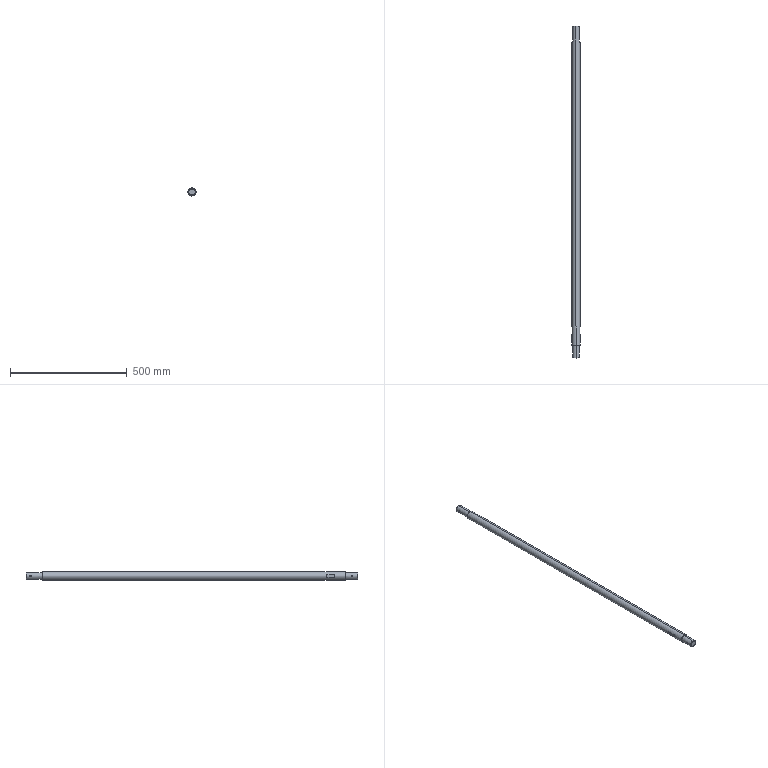Component | SolidWorks | YC1-250-04BalancerAssembly#16673-1_YC1-250-04-06TieRodAxis#16673-1 | 1 solid | 28 faces | box 35 x 1424 x 35 mm | volume 1335790 mm3 | cylinder 10 | plane 10 | cone 8 | commonest cylinder face diameters 30 x4 6 x4 35 x2 | material Plain Carbon Steel
STEP:
#1=COLOUR_RGB('',0.7922,0.8196,0.9333);
#2=FILL_AREA_STYLE_COLOUR('',#1);
#3=FILL_AREA_STYLE('',(#2));
#4=SURFACE_STYLE_FILL_AREA(#3);
#5=SURFACE_SIDE_STYLE('',(#4));
#6=SURFACE_STYLE_USAGE(.BOTH.,#5);
#7=PRESENTATION_STYLE_ASSIGNMENT((#6));
#8=CARTESIAN_POINT('',(-18.689,112.992,-0.1181));
#9=VERTEX_POINT('',#8);
#10=CARTESIAN_POINT('',(-18.689,112.992,0.1181));
#11=VERTEX_POINT('',#10);
#12=CARTESIAN_POINT('',(-18.689,112.992,-0.1181));
#13=CARTESIAN_POINT('',(-18.689,113.,-0.1181));
#14=CARTESIAN_POINT('',(-18.689,113.008,-0.1173));
#15=CARTESIAN_POINT('',(-18.69,113.023,-0.1143));
#16=CARTESIAN_POINT('',(-18.69,113.03,-0.112));
#17=CARTESIAN_POINT('',(-18.691,113.045,-0.1061));
#18=CARTESIAN_POINT('',(-18.692,113.051,-0.1025));
#19=CARTESIAN_POINT('',(-18.693,113.064,-0.09392));
#20=CARTESIAN_POINT('',(-18.694,113.07,-0.08895));
#21=CARTESIAN_POINT('',(-18.696,113.081,-0.07808));
#22=CARTESIAN_POINT('',(-18.696,113.086,-0.07215));
#23=CARTESIAN_POINT('',(-18.698,113.095,-0.05925));
#24=CARTESIAN_POINT('',(-18.699,113.098,-0.05241));
#25=CARTESIAN_POINT('',(-18.7,113.104,-0.03821));
#26=CARTESIAN_POINT('',(-18.7,113.106,-0.03075));
#27=CARTESIAN_POINT('',(-18.701,113.109,-0.01549));
#28=CARTESIAN_POINT('',(-18.701,113.11,-0.007819));
#29=CARTESIAN_POINT('',(-18.701,113.11,0.007627));
#30=CARTESIAN_POINT('',(-18.701,113.109,0.01548));
#31=CARTESIAN_POINT('',(-18.7,113.106,0.03064));
#32=CARTESIAN_POINT('',(-18.7,113.104,0.03801));
#33=CARTESIAN_POINT('',(-18.699,113.098,0.05233));
#34=CARTESIAN_POINT('',(-18.698,113.095,0.05922));
#35=CARTESIAN_POINT('',(-18.696,113.086,0.07199));
#36=CARTESIAN_POINT('',(-18.696,113.081,0.07798));
#37=CARTESIAN_POINT('',(-18.694,113.07,0.08896));
#38=CARTESIAN_POINT('',(-18.693,113.064,0.09384));
#39=CARTESIAN_POINT('',(-18.692,113.051,0.1024));
#40=CARTESIAN_POINT('',(-18.691,113.045,0.1061));
#41=CARTESIAN_POINT('',(-18.69,113.03,0.112));
#42=CARTESIAN_POINT('',(-18.69,113.023,0.1143));
#43=CARTESIAN_POINT('',(-18.689,113.008,0.1173));
#44=CARTESIAN_POINT('',(-18.689,113.,0.1181));
#45=CARTESIAN_POINT('',(-18.689,112.992,0.1181));
#46=B_SPLINE_CURVE_WITH_KNOTS('',3,(#12,#13,#14,#15,#16,#17,#18,#19,#20,#21,#22,#23,#24,#25,#26,#27,#28,#29,#30,#31,#32,#33,#34,#35,#36,#37,#38,#39,#40,#41,#42,#43,#44,#45),.UNSPECIFIED.,.F.,.F.,(4,2,2,2,2,2,2,2,2,2,2,2,2,2,2,2,4),(0.,0.0005875,0.001175,0.001763,0.00235,0.002938,0.003525,0.004113,0.0047,0.005288,0.005875,0.006463,0.00705,0.007638,0.008225,0.008813,0.009401),.UNSPECIFIED.);
#47=EDGE_CURVE('',#9,#11,#46,.T.);
#48=ORIENTED_EDGE('',*,*,#47,.T.);
#49=CARTESIAN_POINT('',(-18.689,112.992,0.1181));
#50=CARTESIAN_POINT('',(-18.689,112.984,0.1181));
#51=CARTESIAN_POINT('',(-18.689,112.977,0.1173));
#52=CARTESIAN_POINT('',(-18.69,112.961,0.1143));
#53=CARTESIAN_POINT('',(-18.69,112.954,0.112));
#54=CARTESIAN_POINT('',(-18.691,112.94,0.1061));
#55=CARTESIAN_POINT('',(-18.692,112.933,0.1025));
#56=CARTESIAN_POINT('',(-18.693,112.92,0.09392));
#57=CARTESIAN_POINT('',(-18.694,112.914,0.08895));
#58=CARTESIAN_POINT('',(-18.696,112.903,0.07808));
#59=CARTESIAN_POINT('',(-18.696,112.898,0.07215));
#60=CARTESIAN_POINT('',(-18.698,112.89,0.05925));
#61=CARTESIAN_POINT('',(-18.699,112.886,0.05241));
#62=CARTESIAN_POINT('',(-18.7,112.88,0.03821));
#63=CARTESIAN_POINT('',(-18.7,112.878,0.03075));
#64=CARTESIAN_POINT('',(-18.701,112.875,0.01549));
#65=CARTESIAN_POINT('',(-18.701,112.874,0.007819));
#66=CARTESIAN_POINT('',(-18.701,112.874,-0.007627));
#67=CARTESIAN_POINT('',(-18.701,112.875,-0.01548));
#68=CARTESIAN_POINT('',(-18.7,112.878,-0.03064));
#69=CARTESIAN_POINT('',(-18.7,112.88,-0.03801));
#70=CARTESIAN_POINT('',(-18.699,112.886,-0.05233));
#71=CARTESIAN_POINT('',(-18.698,112.89,-0.05922));
#72=CARTESIAN_POINT('',(-18.696,112.898,-0.07199));
#73=CARTESIAN_POINT('',(-18.696,112.903,-0.07798));
#74=CARTESIAN_POINT('',(-18.694,112.914,-0.08896));
#75=CARTESIAN_POINT('',(-18.693,112.92,-0.09384));
#76=CARTESIAN_POINT('',(-18.692,112.933,-0.1024));
#77=CARTESIAN_POINT('',(-18.691,112.94,-0.1061));
#78=CARTESIAN_POINT('',(-18.69,112.954,-0.112));
#79=CARTESIAN_POINT('',(-18.69,112.961,-0.1143));
#80=CARTESIAN_POINT('',(-18.689,112.976,-0.1173));
#81=CARTESIAN_POINT('',(-18.689,112.984,-0.1181));
#82=CARTESIAN_POINT('',(-18.689,112.992,-0.1181));
#83=B_SPLINE_CURVE_WITH_KNOTS('',3,(#49,#50,#51,#52,#53,#54,#55,#56,#57,#58,#59,#60,#61,#62,#63,#64,#65,#66,#67,#68,#69,#70,#71,#72,#73,#74,#75,#76,#77,#78,#79,#80,#81,#82),.UNSPECIFIED.,.F.,.F.,(4,2,2,2,2,2,2,2,2,2,2,2,2,2,2,2,4),(0.009401,0.009988,0.01058,0.01116,0.01175,0.01234,0.01293,0.01351,0.0141,0.01469,0.01528,0.01586,0.01645,0.01704,0.01763,0.01821,0.0188),.UNSPECIFIED.);
#84=EDGE_CURVE('',#11,#9,#83,.T.);
#85=ORIENTED_EDGE('',*,*,#84,.T.);
#86=EDGE_LOOP('',(#48,#85));
#87=FACE_BOUND('',#86,.T.);
#88=CARTESIAN_POINT('',(-18.11,114.173,0.5906));
#89=VERTEX_POINT('',#88);
#90=CARTESIAN_POINT('',(-18.11,114.173,-0.5906));
#91=VERTEX_POINT('',#90);
#92=CARTESIAN_POINT('',(-18.11,114.173,0.));
#93=DIRECTION('',(0.,-1.,-0.));
#94=DIRECTION('',(0.,0.,1.));
#95=AXIS2_PLACEMENT_3D('',#92,#93,#94);
#96=CIRCLE('',#95,0.5906);
#97=EDGE_CURVE('',#89,#91,#96,.T.);
#98=ORIENTED_EDGE('',*,*,#97,.T.);
#99=CARTESIAN_POINT('',(-18.11,112.087,-0.5906));
#100=VERTEX_POINT('',#99);
#101=CARTESIAN_POINT('',(-18.11,112.008,-0.5906));
#102=DIRECTION('',(0.,-1.,-0.));
#103=VECTOR('',#102,39.37);
#104=LINE('',#101,#103);
#105=EDGE_CURVE('',#91,#100,#104,.T.);
#106=ORIENTED_EDGE('',*,*,#105,.T.);
#107=CARTESIAN_POINT('',(-18.11,112.087,0.5906));
#108=VERTEX_POINT('',#107);
#109=CARTESIAN_POINT('',(-18.11,112.087,0.));
#110=DIRECTION('',(-0.,1.,0.));
#111=DIRECTION('',(0.,0.,1.));
#112=AXIS2_PLACEMENT_3D('',#109,#110,#111);
#113=CIRCLE('',#112,0.5906);
#114=EDGE_CURVE('',#100,#108,#113,.T.);
#115=ORIENTED_EDGE('',*,*,#114,.T.);
#116=CARTESIAN_POINT('',(-18.11,112.008,0.5906));
#117=DIRECTION('',(0.,-1.,-0.));
#118=VECTOR('',#117,39.37);
#119=LINE('',#116,#118);
#120=EDGE_CURVE('',#89,#108,#119,.T.);
#121=ORIENTED_EDGE('',*,*,#120,.F.);
#122=EDGE_LOOP('',(#98,#106,#115,#121));
#123=FACE_OUTER_BOUND('',#122,.T.);
#124=CARTESIAN_POINT('',(-18.11,112.008,0.));
#125=DIRECTION('',(0.,-1.,-0.));
#126=DIRECTION('',(0.,0.,1.));
#127=AXIS2_PLACEMENT_3D('',#124,#125,#126);
#128=CYLINDRICAL_SURFACE('',#127,0.5906);
#129=ADVANCED_FACE('',(#87,#123),#128,.T.);
#130=ORIENTED_EDGE('',*,*,#84,.F.);
#131=CARTESIAN_POINT('',(-17.532,112.992,0.1181));
#132=VERTEX_POINT('',#131);
#133=CARTESIAN_POINT('',(-17.52,112.992,0.1181));
#134=DIRECTION('',(1.,0.,-0.));
#135=VECTOR('',#134,39.37);
#136=LINE('',#133,#135);
#137=EDGE_CURVE('',#11,#132,#136,.T.);
#138=ORIENTED_EDGE('',*,*,#137,.T.);
#139=CARTESIAN_POINT('',(-17.532,112.992,-0.1181));
#140=VERTEX_POINT('',#139);
#141=CARTESIAN_POINT('',(-17.532,112.992,-0.1181));
#142=CARTESIAN_POINT('',(-17.532,112.984,-0.1181));
#143=CARTESIAN_POINT('',(-17.531,112.977,-0.1173));
#144=CARTESIAN_POINT('',(-17.531,112.961,-0.1143));
#145=CARTESIAN_POINT('',(-17.53,112.954,-0.112));
#146=CARTESIAN_POINT('',(-17.529,112.94,-0.1061));
#147=CARTESIAN_POINT('',(-17.529,112.933,-0.1025));
#148=CARTESIAN_POINT('',(-17.527,112.92,-0.09392));
#149=CARTESIAN_POINT('',(-17.526,112.914,-0.08895));
#150=CARTESIAN_POINT('',(-17.525,112.903,-0.07808));
#151=CARTESIAN_POINT('',(-17.524,112.898,-0.07215));
#152=CARTESIAN_POINT('',(-17.523,112.89,-0.05925));
#153=CARTESIAN_POINT('',(-17.522,112.886,-0.05241));
#154=CARTESIAN_POINT('',(-17.521,112.88,-0.03821));
#155=CARTESIAN_POINT('',(-17.52,112.878,-0.03075));
#156=CARTESIAN_POINT('',(-17.52,112.875,-0.01549));
#157=CARTESIAN_POINT('',(-17.52,112.874,-0.007819));
#158=CARTESIAN_POINT('',(-17.52,112.874,0.007627));
#159=CARTESIAN_POINT('',(-17.52,112.875,0.01548));
#160=CARTESIAN_POINT('',(-17.52,112.878,0.03064));
#161=CARTESIAN_POINT('',(-17.521,112.88,0.03801));
#162=CARTESIAN_POINT('',(-17.522,112.886,0.05233));
#163=CARTESIAN_POINT('',(-17.523,112.89,0.05922));
#164=CARTESIAN_POINT('',(-17.524,112.898,0.07199));
#165=CARTESIAN_POINT('',(-17.525,112.903,0.07798));
#166=CARTESIAN_POINT('',(-17.526,112.914,0.08896));
#167=CARTESIAN_POINT('',(-17.527,112.92,0.09384));
#168=CARTESIAN_POINT('',(-17.529,112.933,0.1024));
#169=CARTESIAN_POINT('',(-17.529,112.94,0.1061));
#170=CARTESIAN_POINT('',(-17.53,112.954,0.112));
#171=CARTESIAN_POINT('',(-17.531,112.961,0.1143));
#172=CARTESIAN_POINT('',(-17.531,112.976,0.1173));
#173=CARTESIAN_POINT('',(-17.532,112.984,0.1181));
#174=CARTESIAN_POINT('',(-17.532,112.992,0.1181));
#175=B_SPLINE_CURVE_WITH_KNOTS('',3,(#141,#142,#143,#144,#145,#146,#147,#148,#149,#150,#151,#152,#153,#154,#155,#156,#157,#158,#159,#160,#161,#162,#163,#164,#165,#166,#167,#168,#169,#170,#171,#172,#173,#174),.UNSPECIFIED.,.F.,.F.,(4,2,2,2,2,2,2,2,2,2,2,2,2,2,2,2,4),(0.,0.0005875,0.001175,0.001763,0.00235,0.002938,0.003525,0.004113,0.0047,0.005288,0.005875,0.006463,0.00705,0.007638,0.008225,0.008813,0.009401),.UNSPECIFIED.);
#176=EDGE_CURVE('',#140,#132,#175,.T.);
#177=ORIENTED_EDGE('',*,*,#176,.F.);
#178=CARTESIAN_POINT('',(-17.52,112.992,-0.1181));
#179=DIRECTION('',(1.,0.,-0.));
#180=VECTOR('',#179,39.37);
#181=LINE('',#178,#180);
#182=EDGE_CURVE('',#9,#140,#181,.T.);
#183=ORIENTED_EDGE('',*,*,#182,.F.);
#184=EDGE_LOOP('',(#130,#138,#177,#183));
#185=FACE_OUTER_BOUND('',#184,.T.);
#186=CARTESIAN_POINT('',(-17.52,112.992,0.));
#187=DIRECTION('',(1.,0.,-0.));
#188=DIRECTION('',(0.,0.,-1.));
#189=AXIS2_PLACEMENT_3D('',#186,#187,#188);
#190=CYLINDRICAL_SURFACE('',#189,0.1181);
#191=ADVANCED_FACE('',(#185),#190,.F.);
#192=CARTESIAN_POINT('',(-18.11,112.008,-0.5118));
#193=VERTEX_POINT('',#192);
#194=CARTESIAN_POINT('',(-18.11,112.008,0.5118));
#195=VERTEX_POINT('',#194);
#196=CARTESIAN_POINT('',(-18.11,112.008,0.));
#197=DIRECTION('',(-0.,1.,0.));
#198=DIRECTION('',(0.,0.,-1.));
#199=AXIS2_PLACEMENT_3D('',#196,#197,#198);
#200=CIRCLE('',#199,0.5118);
#201=EDGE_CURVE('',#193,#195,#200,.T.);
#202=ORIENTED_EDGE('',*,*,#201,.T.);
#203=CARTESIAN_POINT('',(-18.11,112.087,0.5906));
#204=DIRECTION('',(-0.,0.7071,0.7071));
#205=VECTOR('',#204,39.37);
#206=LINE('',#203,#205);
#207=EDGE_CURVE('',#195,#108,#206,.T.);
#208=ORIENTED_EDGE('',*,*,#207,.T.);
#209=ORIENTED_EDGE('',*,*,#114,.F.);
#210=CARTESIAN_POINT('',(-18.11,112.087,-0.5906));
#211=DIRECTION('',(-0.,0.7071,-0.7071));
#212=VECTOR('',#211,39.37);
#213=LINE('',#210,#212);
#214=EDGE_CURVE('',#193,#100,#213,.T.);
#215=ORIENTED_EDGE('',*,*,#214,.F.);
#216=EDGE_LOOP('',(#202,#208,#209,#215));
#217=FACE_OUTER_BOUND('',#216,.T.);
#218=CARTESIAN_POINT('',(-18.11,112.087,0.));
#219=DIRECTION('',(-0.,1.,0.));
#220=DIRECTION('',(0.,0.,-1.));
#221=AXIS2_PLACEMENT_3D('',#218,#219,#220);
#222=CONICAL_SURFACE('',#221,0.5906,0.7854);
#223=ADVANCED_FACE('',(#217),#222,.T.);
#224=CARTESIAN_POINT('',(-18.11,114.173,0.6693));
#225=VERTEX_POINT('',#224);
#226=CARTESIAN_POINT('',(-18.11,114.173,-0.6693));
#227=VERTEX_POINT('',#226);
#228=CARTESIAN_POINT('',(-18.11,114.173,0.));
#229=DIRECTION('',(0.,-1.,-0.));
#230=DIRECTION('',(0.,0.,1.));
#231=AXIS2_PLACEMENT_3D('',#228,#229,#230);
#232=CIRCLE('',#231,0.6693);
#233=EDGE_CURVE('',#225,#227,#232,.T.);
#234=ORIENTED_EDGE('',*,*,#233,.F.);
#235=CARTESIAN_POINT('',(-18.11,114.193,0.689));
#236=VERTEX_POINT('',#235);
#237=CARTESIAN_POINT('',(-18.11,114.193,0.689));
#238=DIRECTION('',(-0.,0.7071,0.7071));
#239=VECTOR('',#238,39.37);
#240=LINE('',#237,#239);
#241=EDGE_CURVE('',#225,#236,#240,.T.);
#242=ORIENTED_EDGE('',*,*,#241,.T.);
#243=CARTESIAN_POINT('',(-18.11,114.193,-0.689));
#244=VERTEX_POINT('',#243);
#245=CARTESIAN_POINT('',(-18.11,114.193,0.));
#246=DIRECTION('',(0.,-1.,-0.));
#247=DIRECTION('',(0.,0.,1.));
#248=AXIS2_PLACEMENT_3D('',#245,#246,#247);
#249=CIRCLE('',#248,0.689);
#250=EDGE_CURVE('',#236,#244,#249,.T.);
#251=ORIENTED_EDGE('',*,*,#250,.T.);
#252=CARTESIAN_POINT('',(-18.11,114.193,-0.689));
#253=DIRECTION('',(-0.,0.7071,-0.7071));
#254=VECTOR('',#253,39.37);
#255=LINE('',#252,#254);
#256=EDGE_CURVE('',#227,#244,#255,.T.);
#257=ORIENTED_EDGE('',*,*,#256,.F.);
#258=EDGE_LOOP('',(#234,#242,#251,#257));
#259=FACE_OUTER_BOUND('',#258,.T.);
#260=CARTESIAN_POINT('',(-18.11,114.193,0.));
#261=DIRECTION('',(-0.,1.,0.));
#262=DIRECTION('',(0.,0.,-1.));
#263=AXIS2_PLACEMENT_3D('',#260,#261,#262);
#264=CONICAL_SURFACE('',#263,0.689,0.7854);
#265=ADVANCED_FACE('',(#259),#264,.T.);
#266=CARTESIAN_POINT('',(-18.76,115.945,-0.2296));
#267=VERTEX_POINT('',#266);
#268=CARTESIAN_POINT('',(-18.76,117.283,-0.2296));
#269=VERTEX_POINT('',#268);
#270=CARTESIAN_POINT('',(-18.76,112.008,-0.2296));
#271=DIRECTION('',(-0.,1.,0.));
#272=VECTOR('',#271,39.37);
#273=LINE('',#270,#272);
#274=EDGE_CURVE('',#267,#269,#273,.T.);
#275=ORIENTED_EDGE('',*,*,#274,.T.);
#276=CARTESIAN_POINT('',(-18.76,117.283,0.2296));
#277=VERTEX_POINT('',#276);
#278=CARTESIAN_POINT('',(-18.11,117.283,0.));
#279=DIRECTION('',(-0.,1.,0.));
#280=DIRECTION('',(-0.,0.,1.));
#281=AXIS2_PLACEMENT_3D('',#278,#279,#280);
#282=CIRCLE('',#281,0.689);
#283=EDGE_CURVE('',#269,#277,#282,.T.);
#284=ORIENTED_EDGE('',*,*,#283,.T.);
#285=CARTESIAN_POINT('',(-18.76,115.945,0.2296));
#286=VERTEX_POINT('',#285);
#287=CARTESIAN_POINT('',(-18.76,112.008,0.2296));
#288=DIRECTION('',(0.,-1.,-0.));
#289=VECTOR('',#288,39.37);
#290=LINE('',#287,#289);
#291=EDGE_CURVE('',#277,#286,#290,.T.);
#292=ORIENTED_EDGE('',*,*,#291,.T.);
#293=CARTESIAN_POINT('',(-18.11,115.945,0.));
#294=DIRECTION('',(0.,-1.,-0.));
#295=DIRECTION('',(0.,0.,1.));
#296=AXIS2_PLACEMENT_3D('',#293,#294,#295);
#297=CIRCLE('',#296,0.689);
#298=EDGE_CURVE('',#286,#267,#297,.T.);
#299=ORIENTED_EDGE('',*,*,#298,.T.);
#300=EDGE_LOOP('',(#275,#284,#292,#299));
#301=FACE_BOUND('',#300,.T.);
#302=CARTESIAN_POINT('',(-18.11,165.335,0.689));
#303=VERTEX_POINT('',#302);
#304=CARTESIAN_POINT('',(-18.11,165.335,-0.689));
#305=VERTEX_POINT('',#304);
#306=CARTESIAN_POINT('',(-18.11,165.335,0.));
#307=DIRECTION('',(0.,-1.,-0.));
#308=DIRECTION('',(0.,0.,1.));
#309=AXIS2_PLACEMENT_3D('',#306,#307,#308);
#310=CIRCLE('',#309,0.689);
#311=EDGE_CURVE('',#303,#305,#310,.T.);
#312=ORIENTED_EDGE('',*,*,#311,.T.);
#313=CARTESIAN_POINT('',(-18.11,112.008,-0.689));
#314=DIRECTION('',(0.,-1.,-0.));
#315=VECTOR('',#314,39.37);
#316=LINE('',#313,#315);
#317=EDGE_CURVE('',#305,#244,#316,.T.);
#318=ORIENTED_EDGE('',*,*,#317,.T.);
#319=ORIENTED_EDGE('',*,*,#250,.F.);
#320=CARTESIAN_POINT('',(-18.11,112.008,0.689));
#321=DIRECTION('',(0.,-1.,-0.));
#322=VECTOR('',#321,39.37);
#323=LINE('',#320,#322);
#324=EDGE_CURVE('',#303,#236,#323,.T.);
#325=ORIENTED_EDGE('',*,*,#324,.F.);
#326=EDGE_LOOP('',(#312,#318,#319,#325));
#327=FACE_OUTER_BOUND('',#326,.T.);
#328=CARTESIAN_POINT('',(-18.11,112.008,0.));
#329=DIRECTION('',(0.,-1.,-0.));
#330=DIRECTION('',(0.,0.,1.));
#331=AXIS2_PLACEMENT_3D('',#328,#329,#330);
#332=CYLINDRICAL_SURFACE('',#331,0.689);
#333=ADVANCED_FACE('',(#301,#327),#332,.T.);
#334=CARTESIAN_POINT('',(-18.11,165.354,0.6693));
#335=VERTEX_POINT('',#334);
#336=CARTESIAN_POINT('',(-18.11,165.354,-0.6693));
#337=VERTEX_POINT('',#336);
#338=CARTESIAN_POINT('',(-18.11,165.354,0.));
#339=DIRECTION('',(0.,-1.,-0.));
#340=DIRECTION('',(0.,0.,1.));
#341=AXIS2_PLACEMENT_3D('',#338,#339,#340);
#342=CIRCLE('',#341,0.6693);
#343=EDGE_CURVE('',#335,#337,#342,.T.);
#344=ORIENTED_EDGE('',*,*,#343,.T.);
#345=CARTESIAN_POINT('',(-18.11,165.335,-0.689));
#346=DIRECTION('',(0.,-0.7071,-0.7071));
#347=VECTOR('',#346,39.37);
#348=LINE('',#345,#347);
#349=EDGE_CURVE('',#337,#305,#348,.T.);
#350=ORIENTED_EDGE('',*,*,#349,.T.);
#351=ORIENTED_EDGE('',*,*,#311,.F.);
#352=CARTESIAN_POINT('',(-18.11,165.335,0.689));
#353=DIRECTION('',(0.,-0.7071,0.7071));
#354=VECTOR('',#353,39.37);
#355=LINE('',#352,#354);
#356=EDGE_CURVE('',#335,#303,#355,.T.);
#357=ORIENTED_EDGE('',*,*,#356,.F.);
#358=EDGE_LOOP('',(#344,#350,#351,#357));
#359=FACE_OUTER_BOUND('',#358,.T.);
#360=CARTESIAN_POINT('',(-18.11,165.335,0.));
#361=DIRECTION('',(0.,-1.,-0.));
#362=DIRECTION('',(0.,0.,1.));
#363=AXIS2_PLACEMENT_3D('',#360,#361,#362);
#364=CONICAL_SURFACE('',#363,0.689,0.7854);
#365=ADVANCED_FACE('',(#359),#364,.T.);
#366=CARTESIAN_POINT('',(-18.689,167.283,-0.1181));
#367=VERTEX_POINT('',#366);
#368=CARTESIAN_POINT('',(-18.689,167.283,0.1181));
#369=VERTEX_POINT('',#368);
#370=CARTESIAN_POINT('',(-18.689,167.283,-0.1181));
#371=CARTESIAN_POINT('',(-18.689,167.291,-0.1181));
#372=CARTESIAN_POINT('',(-18.689,167.299,-0.1173));
#373=CARTESIAN_POINT('',(-18.69,167.314,-0.1143));
#374=CARTESIAN_POINT('',(-18.69,167.322,-0.112));
#375=CARTESIAN_POINT('',(-18.691,167.336,-0.1061));
#376=CARTESIAN_POINT('',(-18.692,167.343,-0.1025));
#377=CARTESIAN_POINT('',(-18.693,167.355,-0.09392));
#378=CARTESIAN_POINT('',(-18.694,167.362,-0.08895));
#379=CARTESIAN_POINT('',(-18.696,167.372,-0.07808));
#380=CARTESIAN_POINT('',(-18.696,167.377,-0.07215));
#381=CARTESIAN_POINT('',(-18.698,167.386,-0.05925));
#382=CARTESIAN_POINT('',(-18.699,167.39,-0.05241));
#383=CARTESIAN_POINT('',(-18.7,167.395,-0.03821));
#384=CARTESIAN_POINT('',(-18.7,167.398,-0.03075));
#385=CARTESIAN_POINT('',(-18.701,167.401,-0.01549));
#386=CARTESIAN_POINT('',(-18.701,167.402,-0.007819));
#387=CARTESIAN_POINT('',(-18.701,167.402,0.007627));
#388=CARTESIAN_POINT('',(-18.701,167.401,0.01548));
#389=CARTESIAN_POINT('',(-18.7,167.398,0.03064));
#390=CARTESIAN_POINT('',(-18.7,167.396,0.03801));
#391=CARTESIAN_POINT('',(-18.699,167.39,0.05233));
#392=CARTESIAN_POINT('',(-18.698,167.386,0.05922));
#393=CARTESIAN_POINT('',(-18.696,167.377,0.07199));
#394=CARTESIAN_POINT('',(-18.696,167.373,0.07798));
#395=CARTESIAN_POINT('',(-18.694,167.362,0.08896));
#396=CARTESIAN_POINT('',(-18.693,167.356,0.09384));
#397=CARTESIAN_POINT('',(-18.692,167.343,0.1024));
#398=CARTESIAN_POINT('',(-18.691,167.336,0.1061));
#399=CARTESIAN_POINT('',(-18.69,167.322,0.112));
#400=CARTESIAN_POINT('',(-18.69,167.314,0.1143));
#401=CARTESIAN_POINT('',(-18.689,167.299,0.1173));
#402=CARTESIAN_POINT('',(-18.689,167.291,0.1181));
#403=CARTESIAN_POINT('',(-18.689,167.283,0.1181));
#404=B_SPLINE_CURVE_WITH_KNOTS('',3,(#370,#371,#372,#373,#374,#375,#376,#377,#378,#379,#380,#381,#382,#383,#384,#385,#386,#387,#388,#389,#390,#391,#392,#393,#394,#395,#396,#397,#398,#399,#400,#401,#402,#403),.UNSPECIFIED.,.F.,.F.,(4,2,2,2,2,2,2,2,2,2,2,2,2,2,2,2,4),(0.,0.0005875,0.001175,0.001763,0.00235,0.002938,0.003525,0.004113,0.0047,0.005288,0.005875,0.006463,0.00705,0.007638,0.008225,0.008813,0.009401),.UNSPECIFIED.);
#405=EDGE_CURVE('',#367,#369,#404,.T.);
#406=ORIENTED_EDGE('',*,*,#405,.T.);
#407=CARTESIAN_POINT('',(-18.689,167.283,0.1181));
#408=CARTESIAN_POINT('',(-18.689,167.276,0.1181));
#409=CARTESIAN_POINT('',(-18.689,167.268,0.1173));
#410=CARTESIAN_POINT('',(-18.69,167.253,0.1143));
#411=CARTESIAN_POINT('',(-18.69,167.245,0.112));
#412=CARTESIAN_POINT('',(-18.691,167.231,0.1061));
#413=CARTESIAN_POINT('',(-18.692,167.224,0.1025));
#414=CARTESIAN_POINT('',(-18.693,167.211,0.09392));
#415=CARTESIAN_POINT('',(-18.694,167.205,0.08895));
#416=CARTESIAN_POINT('',(-18.696,167.195,0.07808));
#417=CARTESIAN_POINT('',(-18.696,167.19,0.07215));
#418=CARTESIAN_POINT('',(-18.698,167.181,0.05925));
#419=CARTESIAN_POINT('',(-18.699,167.177,0.05241));
#420=CARTESIAN_POINT('',(-18.7,167.171,0.03821));
#421=CARTESIAN_POINT('',(-18.7,167.169,0.03075));
#422=CARTESIAN_POINT('',(-18.701,167.166,0.01549));
#423=CARTESIAN_POINT('',(-18.701,167.165,0.007819));
#424=CARTESIAN_POINT('',(-18.701,167.165,-0.007627));
#425=CARTESIAN_POINT('',(-18.701,167.166,-0.01548));
#426=CARTESIAN_POINT('',(-18.7,167.169,-0.03064));
#427=CARTESIAN_POINT('',(-18.7,167.171,-0.03801));
#428=CARTESIAN_POINT('',(-18.699,167.177,-0.05233));
#429=CARTESIAN_POINT('',(-18.698,167.181,-0.05922));
#430=CARTESIAN_POINT('',(-18.696,167.19,-0.07199));
#431=CARTESIAN_POINT('',(-18.696,167.194,-0.07798));
#432=CARTESIAN_POINT('',(-18.694,167.205,-0.08896));
#433=CARTESIAN_POINT('',(-18.693,167.211,-0.09384));
#434=CARTESIAN_POINT('',(-18.692,167.224,-0.1024));
#435=CARTESIAN_POINT('',(-18.691,167.231,-0.1061));
#436=CARTESIAN_POINT('',(-18.69,167.245,-0.112));
#437=CARTESIAN_POINT('',(-18.69,167.253,-0.1143));
#438=CARTESIAN_POINT('',(-18.689,167.268,-0.1173));
#439=CARTESIAN_POINT('',(-18.689,167.276,-0.1181));
#440=CARTESIAN_POINT('',(-18.689,167.283,-0.1181));
#441=B_SPLINE_CURVE_WITH_KNOTS('',3,(#407,#408,#409,#410,#411,#412,#413,#414,#415,#416,#417,#418,#419,#420,#421,#422,#423,#424,#425,#426,#427,#428,#429,#430,#431,#432,#433,#434,#435,#436,#437,#438,#439,#440),.UNSPECIFIED.,.F.,.F.,(4,2,2,2,2,2,2,2,2,2,2,2,2,2,2,2,4),(0.009401,0.009988,0.01058,0.01116,0.01175,0.01234,0.01293,0.01351,0.0141,0.01469,0.01528,0.01586,0.01645,0.01704,0.01763,0.01821,0.0188),.UNSPECIFIED.);
#442=EDGE_CURVE('',#369,#367,#441,.T.);
#443=ORIENTED_EDGE('',*,*,#442,.T.);
#444=EDGE_LOOP('',(#406,#443));
#445=FACE_BOUND('',#444,.T.);
#446=CARTESIAN_POINT('',(-18.11,167.992,0.5906));
#447=VERTEX_POINT('',#446);
#448=CARTESIAN_POINT('',(-18.11,167.992,-0.5906));
#449=VERTEX_POINT('',#448);
#450=CARTESIAN_POINT('',(-18.11,167.992,0.));
#451=DIRECTION('',(0.,-1.,-0.));
#452=DIRECTION('',(0.,0.,1.));
#453=AXIS2_PLACEMENT_3D('',#450,#451,#452);
#454=CIRCLE('',#453,0.5906);
#455=EDGE_CURVE('',#447,#449,#454,.T.);
#456=ORIENTED_EDGE('',*,*,#455,.T.);
#457=CARTESIAN_POINT('',(-18.11,165.354,-0.5906));
#458=VERTEX_POINT('',#457);
#459=CARTESIAN_POINT('',(-18.11,112.008,-0.5906));
#460=DIRECTION('',(0.,-1.,-0.));
#461=VECTOR('',#460,39.37);
#462=LINE('',#459,#461);
#463=EDGE_CURVE('',#449,#458,#462,.T.);
#464=ORIENTED_EDGE('',*,*,#463,.T.);
#465=CARTESIAN_POINT('',(-18.11,165.354,0.5906));
#466=VERTEX_POINT('',#465);
#467=CARTESIAN_POINT('',(-18.11,165.354,0.));
#468=DIRECTION('',(0.,-1.,-0.));
#469=DIRECTION('',(0.,0.,1.));
#470=AXIS2_PLACEMENT_3D('',#467,#468,#469);
#471=CIRCLE('',#470,0.5906);
#472=EDGE_CURVE('',#466,#458,#471,.T.);
#473=ORIENTED_EDGE('',*,*,#472,.F.);
#474=CARTESIAN_POINT('',(-18.11,112.008,0.5906));
#475=DIRECTION('',(0.,-1.,-0.));
#476=VECTOR('',#475,39.37);
#477=LINE('',#474,#476);
#478=EDGE_CURVE('',#447,#466,#477,.T.);
#479=ORIENTED_EDGE('',*,*,#478,.F.);
#480=EDGE_LOOP('',(#456,#464,#473,#479));
#481=FACE_OUTER_BOUND('',#480,.T.);
#482=CARTESIAN_POINT('',(-18.11,112.008,0.));
#483=DIRECTION('',(0.,-1.,-0.));
#484=DIRECTION('',(0.,0.,1.));
#485=AXIS2_PLACEMENT_3D('',#482,#483,#484);
#486=CYLINDRICAL_SURFACE('',#485,0.5906);
#487=ADVANCED_FACE('',(#445,#481),#486,.T.);
#488=ORIENTED_EDGE('',*,*,#442,.F.);
#489=CARTESIAN_POINT('',(-17.532,167.283,0.1181));
#490=VERTEX_POINT('',#489);
#491=CARTESIAN_POINT('',(-17.52,167.283,0.1181));
#492=DIRECTION('',(1.,0.,-0.));
#493=VECTOR('',#492,39.37);
#494=LINE('',#491,#493);
#495=EDGE_CURVE('',#369,#490,#494,.T.);
#496=ORIENTED_EDGE('',*,*,#495,.T.);
#497=CARTESIAN_POINT('',(-17.532,167.283,-0.1181));
#498=VERTEX_POINT('',#497);
#499=CARTESIAN_POINT('',(-17.532,167.283,-0.1181));
#500=CARTESIAN_POINT('',(-17.532,167.276,-0.1181));
#501=CARTESIAN_POINT('',(-17.531,167.268,-0.1173));
#502=CARTESIAN_POINT('',(-17.531,167.253,-0.1143));
#503=CARTESIAN_POINT('',(-17.53,167.245,-0.112));
#504=CARTESIAN_POINT('',(-17.529,167.231,-0.1061));
#505=CARTESIAN_POINT('',(-17.529,167.224,-0.1025));
#506=CARTESIAN_POINT('',(-17.527,167.211,-0.09392));
#507=CARTESIAN_POINT('',(-17.526,167.205,-0.08895));
#508=CARTESIAN_POINT('',(-17.525,167.195,-0.07808));
#509=CARTESIAN_POINT('',(-17.524,167.19,-0.07215));
#510=CARTESIAN_POINT('',(-17.523,167.181,-0.05925));
#511=CARTESIAN_POINT('',(-17.522,167.177,-0.05241));
#512=CARTESIAN_POINT('',(-17.521,167.171,-0.03821));
#513=CARTESIAN_POINT('',(-17.52,167.169,-0.03075));
#514=CARTESIAN_POINT('',(-17.52,167.166,-0.01549));
#515=CARTESIAN_POINT('',(-17.52,167.165,-0.007819));
#516=CARTESIAN_POINT('',(-17.52,167.165,0.007627));
#517=CARTESIAN_POINT('',(-17.52,167.166,0.01548));
#518=CARTESIAN_POINT('',(-17.52,167.169,0.03064));
#519=CARTESIAN_POINT('',(-17.521,167.171,0.03801));
#520=CARTESIAN_POINT('',(-17.522,167.177,0.05233));
#521=CARTESIAN_POINT('',(-17.523,167.181,0.05922));
#522=CARTESIAN_POINT('',(-17.524,167.19,0.07199));
#523=CARTESIAN_POINT('',(-17.525,167.194,0.07798));
#524=CARTESIAN_POINT('',(-17.526,167.205,0.08896));
#525=CARTESIAN_POINT('',(-17.527,167.211,0.09384));
#526=CARTESIAN_POINT('',(-17.529,167.224,0.1024));
#527=CARTESIAN_POINT('',(-17.529,167.231,0.1061));
#528=CARTESIAN_POINT('',(-17.53,167.245,0.112));
#529=CARTESIAN_POINT('',(-17.531,167.253,0.1143));
#530=CARTESIAN_POINT('',(-17.531,167.268,0.1173));
#531=CARTESIAN_POINT('',(-17.532,167.276,0.1181));
#532=CARTESIAN_POINT('',(-17.532,167.283,0.1181));
#533=B_SPLINE_CURVE_WITH_KNOTS('',3,(#499,#500,#501,#502,#503,#504,#505,#506,#507,#508,#509,#510,#511,#512,#513,#514,#515,#516,#517,#518,#519,#520,#521,#522,#523,#524,#525,#526,#527,#528,#529,#530,#531,#532),.UNSPECIFIED.,.F.,.F.,(4,2,2,2,2,2,2,2,2,2,2,2,2,2,2,2,4),(0.,0.0005875,0.001175,0.001763,0.00235,0.002938,0.003525,0.004113,0.0047,0.005288,0.005875,0.006463,0.00705,0.007638,0.008225,0.008813,0.009401),.UNSPECIFIED.);
#534=EDGE_CURVE('',#498,#490,#533,.T.);
#535=ORIENTED_EDGE('',*,*,#534,.F.);
#536=CARTESIAN_POINT('',(-17.52,167.283,-0.1181));
#537=DIRECTION('',(1.,0.,-0.));
#538=VECTOR('',#537,39.37);
#539=LINE('',#536,#538);
#540=EDGE_CURVE('',#367,#498,#539,.T.);
#541=ORIENTED_EDGE('',*,*,#540,.F.);
#542=EDGE_LOOP('',(#488,#496,#535,#541));
#543=FACE_OUTER_BOUND('',#542,.T.);
#544=CARTESIAN_POINT('',(-17.52,167.283,0.));
#545=DIRECTION('',(1.,0.,-0.));
#546=DIRECTION('',(0.,0.,-1.));
#547=AXIS2_PLACEMENT_3D('',#544,#545,#546);
#548=CYLINDRICAL_SURFACE('',#547,0.1181);
#549=ADVANCED_FACE('',(#543),#548,.F.);
#550=CARTESIAN_POINT('',(-18.11,168.071,0.5118));
#551=VERTEX_POINT('',#550);
#552=CARTESIAN_POINT('',(-18.11,168.071,-0.5118));
#553=VERTEX_POINT('',#552);
#554=CARTESIAN_POINT('',(-18.11,168.071,0.));
#555=DIRECTION('',(0.,-1.,-0.));
#556=DIRECTION('',(0.,0.,1.));
#557=AXIS2_PLACEMENT_3D('',#554,#555,#556);
#558=CIRCLE('',#557,0.5118);
#559=EDGE_CURVE('',#551,#553,#558,.T.);
#560=ORIENTED_EDGE('',*,*,#559,.T.);
#561=CARTESIAN_POINT('',(-18.11,167.992,-0.5906));
#562=DIRECTION('',(0.,-0.7071,-0.7071));
#563=VECTOR('',#562,39.37);
#564=LINE('',#561,#563);
#565=EDGE_CURVE('',#553,#449,#564,.T.);
#566=ORIENTED_EDGE('',*,*,#565,.T.);
#567=ORIENTED_EDGE('',*,*,#455,.F.);
#568=CARTESIAN_POINT('',(-18.11,167.992,0.5906));
#569=DIRECTION('',(0.,-0.7071,0.7071));
#570=VECTOR('',#569,39.37);
#571=LINE('',#568,#570);
#572=EDGE_CURVE('',#551,#447,#571,.T.);
#573=ORIENTED_EDGE('',*,*,#572,.F.);
#574=EDGE_LOOP('',(#560,#566,#567,#573));
#575=FACE_OUTER_BOUND('',#574,.T.);
#576=CARTESIAN_POINT('',(-18.11,167.992,0.));
#577=DIRECTION('',(0.,-1.,-0.));
#578=DIRECTION('',(0.,0.,1.));
#579=AXIS2_PLACEMENT_3D('',#576,#577,#578);
#580=CONICAL_SURFACE('',#579,0.5906,0.7854);
#581=ADVANCED_FACE('',(#575),#580,.T.);
#582=ORIENTED_EDGE('',*,*,#317,.F.);
#583=CARTESIAN_POINT('',(-18.11,165.335,0.));
#584=DIRECTION('',(0.,-1.,-0.));
#585=DIRECTION('',(0.,0.,1.));
#586=AXIS2_PLACEMENT_3D('',#583,#584,#585);
#587=CIRCLE('',#586,0.689);
#588=EDGE_CURVE('',#305,#303,#587,.T.);
#589=ORIENTED_EDGE('',*,*,#588,.T.);
#590=ORIENTED_EDGE('',*,*,#324,.T.);
#591=CARTESIAN_POINT('',(-18.11,114.193,0.));
#592=DIRECTION('',(0.,-1.,-0.));
#593=DIRECTION('',(0.,0.,1.));
#594=AXIS2_PLACEMENT_3D('',#591,#592,#593);
#595=CIRCLE('',#594,0.689);
#596=EDGE_CURVE('',#244,#236,#595,.T.);
#597=ORIENTED_EDGE('',*,*,#596,.F.);
#598=EDGE_LOOP('',(#582,#589,#590,#597));
#599=FACE_OUTER_BOUND('',#598,.T.);
#600=CARTESIAN_POINT('',(-17.461,115.945,-0.2296));
#601=VERTEX_POINT('',#600);
#602=CARTESIAN_POINT('',(-17.461,115.945,0.2296));
#603=VERTEX_POINT('',#602);
#604=CARTESIAN_POINT('',(-18.11,115.945,0.));
#605=DIRECTION('',(0.,-1.,-0.));
#606=DIRECTION('',(0.,0.,1.));
#607=AXIS2_PLACEMENT_3D('',#604,#605,#606);
#608=CIRCLE('',#607,0.689);
#609=EDGE_CURVE('',#601,#603,#608,.T.);
#610=ORIENTED_EDGE('',*,*,#609,.T.);
#611=CARTESIAN_POINT('',(-17.461,117.283,0.2296));
#612=VERTEX_POINT('',#611);
#613=CARTESIAN_POINT('',(-17.461,112.008,0.2296));
#614=DIRECTION('',(-0.,1.,0.));
#615=VECTOR('',#614,39.37);
#616=LINE('',#613,#615);
#617=EDGE_CURVE('',#603,#612,#616,.T.);
#618=ORIENTED_EDGE('',*,*,#617,.T.);
#619=CARTESIAN_POINT('',(-17.461,117.283,-0.2296));
#620=VERTEX_POINT('',#619);
#621=CARTESIAN_POINT('',(-18.11,117.283,0.));
#622=DIRECTION('',(-0.,1.,0.));
#623=DIRECTION('',(-0.,0.,1.));
#624=AXIS2_PLACEMENT_3D('',#621,#622,#623);
#625=CIRCLE('',#624,0.689);
#626=EDGE_CURVE('',#612,#620,#625,.T.);
#627=ORIENTED_EDGE('',*,*,#626,.T.);
#628=CARTESIAN_POINT('',(-17.461,112.008,-0.2296));
#629=DIRECTION('',(0.,-1.,-0.));
#630=VECTOR('',#629,39.37);
#631=LINE('',#628,#630);
#632=EDGE_CURVE('',#620,#601,#631,.T.);
#633=ORIENTED_EDGE('',*,*,#632,.T.);
#634=EDGE_LOOP('',(#610,#618,#627,#633));
#635=FACE_BOUND('',#634,.T.);
#636=CARTESIAN_POINT('',(-18.11,112.008,0.));
#637=DIRECTION('',(0.,-1.,-0.));
#638=DIRECTION('',(0.,0.,1.));
#639=AXIS2_PLACEMENT_3D('',#636,#637,#638);
#640=CYLINDRICAL_SURFACE('',#639,0.689);
#641=ADVANCED_FACE('',(#599,#635),#640,.T.);
#642=ORIENTED_EDGE('',*,*,#349,.F.);
#643=CARTESIAN_POINT('',(-18.11,165.354,0.));
#644=DIRECTION('',(0.,-1.,-0.));
#645=DIRECTION('',(0.,0.,1.));
#646=AXIS2_PLACEMENT_3D('',#643,#644,#645);
#647=CIRCLE('',#646,0.6693);
#648=EDGE_CURVE('',#337,#335,#647,.T.);
#649=ORIENTED_EDGE('',*,*,#648,.T.);
#650=ORIENTED_EDGE('',*,*,#356,.T.);
#651=ORIENTED_EDGE('',*,*,#588,.F.);
#652=EDGE_LOOP('',(#642,#649,#650,#651));
#653=FACE_OUTER_BOUND('',#652,.T.);
#654=CARTESIAN_POINT('',(-18.11,165.335,0.));
#655=DIRECTION('',(0.,-1.,-0.));
#656=DIRECTION('',(0.,0.,1.));
#657=AXIS2_PLACEMENT_3D('',#654,#655,#656);
#658=CONICAL_SURFACE('',#657,0.689,0.7854);
#659=ADVANCED_FACE('',(#653),#658,.T.);
#660=ORIENTED_EDGE('',*,*,#283,.F.);
#661=CARTESIAN_POINT('',(-18.76,117.283,1.969));
#662=DIRECTION('',(0.,0.,-1.));
#663=VECTOR('',#662,39.37);
#664=LINE('',#661,#663);
#665=EDGE_CURVE('',#277,#269,#664,.T.);
#666=ORIENTED_EDGE('',*,*,#665,.F.);
#667=EDGE_LOOP('',(#660,#666));
#668=FACE_OUTER_BOUND('',#667,.T.);
#669=CARTESIAN_POINT('',(-18.799,117.283,1.969));
#670=DIRECTION('',(-0.,1.,0.));
#671=DIRECTION('',(0.,0.,-1.));
#672=AXIS2_PLACEMENT_3D('',#669,#670,#671);
#673=PLANE('',#672);
#674=ADVANCED_FACE('',(#668),#673,.F.);
#675=ORIENTED_EDGE('',*,*,#665,.T.);
#676=ORIENTED_EDGE('',*,*,#274,.F.);
#677=CARTESIAN_POINT('',(-18.76,115.945,1.969));
#678=DIRECTION('',(0.,0.,-1.));
#679=VECTOR('',#678,39.37);
#680=LINE('',#677,#679);
#681=EDGE_CURVE('',#286,#267,#680,.T.);
#682=ORIENTED_EDGE('',*,*,#681,.F.);
#683=ORIENTED_EDGE('',*,*,#291,.F.);
#684=EDGE_LOOP('',(#675,#676,#682,#683));
#685=FACE_OUTER_BOUND('',#684,.T.);
#686=CARTESIAN_POINT('',(-18.76,117.283,1.969));
#687=DIRECTION('',(1.,0.,0.));
#688=DIRECTION('',(0.,-1.,-0.));
#689=AXIS2_PLACEMENT_3D('',#686,#687,#688);
#690=PLANE('',#689);
#691=ADVANCED_FACE('',(#685),#690,.F.);
#692=ORIENTED_EDGE('',*,*,#681,.T.);
#693=ORIENTED_EDGE('',*,*,#298,.F.);
#694=EDGE_LOOP('',(#692,#693));
#695=FACE_OUTER_BOUND('',#694,.T.);
#696=CARTESIAN_POINT('',(-18.799,115.945,1.969));
#697=DIRECTION('',(0.,-1.,-0.));
#698=DIRECTION('',(-0.,-0.,1.));
#699=AXIS2_PLACEMENT_3D('',#696,#697,#698);
#700=PLANE('',#699);
#701=ADVANCED_FACE('',(#695),#700,.F.);
#702=CARTESIAN_POINT('',(-17.461,117.283,1.969));
#703=DIRECTION('',(0.,0.,-1.));
#704=VECTOR('',#703,39.37);
#705=LINE('',#702,#704);
#706=EDGE_CURVE('',#612,#620,#705,.T.);
#707=ORIENTED_EDGE('',*,*,#706,.F.);
#708=ORIENTED_EDGE('',*,*,#617,.F.);
#709=CARTESIAN_POINT('',(-17.461,115.945,1.969));
#710=DIRECTION('',(-0.,-0.,1.));
#711=VECTOR('',#710,39.37);
#712=LINE('',#709,#711);
#713=EDGE_CURVE('',#601,#603,#712,.T.);
#714=ORIENTED_EDGE('',*,*,#713,.F.);
#715=ORIENTED_EDGE('',*,*,#632,.F.);
#716=EDGE_LOOP('',(#707,#708,#714,#715));
#717=FACE_OUTER_BOUND('',#716,.T.);
#718=CARTESIAN_POINT('',(-17.461,117.283,1.969));
#719=DIRECTION('',(-1.,-0.,-0.));
#720=DIRECTION('',(-0.,1.,0.));
#721=AXIS2_PLACEMENT_3D('',#718,#719,#720);
#722=PLANE('',#721);
#723=ADVANCED_FACE('',(#717),#722,.F.);
#724=ORIENTED_EDGE('',*,*,#609,.F.);
#725=ORIENTED_EDGE('',*,*,#713,.T.);
#726=EDGE_LOOP('',(#724,#725));
#727=FACE_OUTER_BOUND('',#726,.T.);
#728=CARTESIAN_POINT('',(-17.421,115.945,1.969));
#729=DIRECTION('',(0.,-1.,-0.));
#730=DIRECTION('',(-0.,-0.,1.));
#731=AXIS2_PLACEMENT_3D('',#728,#729,#730);
#732=PLANE('',#731);
#733=ADVANCED_FACE('',(#727),#732,.F.);
#734=ORIENTED_EDGE('',*,*,#626,.F.);
#735=ORIENTED_EDGE('',*,*,#706,.T.);
#736=EDGE_LOOP('',(#734,#735));
#737=FACE_OUTER_BOUND('',#736,.T.);
#738=CARTESIAN_POINT('',(-17.421,117.283,1.969));
#739=DIRECTION('',(-0.,1.,0.));
#740=DIRECTION('',(0.,0.,-1.));
#741=AXIS2_PLACEMENT_3D('',#738,#739,#740);
#742=PLANE('',#741);
#743=ADVANCED_FACE('',(#737),#742,.F.);
#744=ORIENTED_EDGE('',*,*,#472,.T.);
#745=CARTESIAN_POINT('',(-18.11,165.354,0.));
#746=DIRECTION('',(0.,-1.,-0.));
#747=DIRECTION('',(0.,0.,1.));
#748=AXIS2_PLACEMENT_3D('',#745,#746,#747);
#749=CIRCLE('',#748,0.5906);
#750=EDGE_CURVE('',#458,#466,#749,.T.);
#751=ORIENTED_EDGE('',*,*,#750,.T.);
#752=EDGE_LOOP('',(#744,#751));
#753=FACE_BOUND('',#752,.T.);
#754=ORIENTED_EDGE('',*,*,#343,.F.);
#755=ORIENTED_EDGE('',*,*,#648,.F.);
#756=EDGE_LOOP('',(#754,#755));
#757=FACE_OUTER_BOUND('',#756,.T.);
#758=CARTESIAN_POINT('',(-18.701,165.354,0.));
#759=DIRECTION('',(-0.,1.,0.));
#760=DIRECTION('',(0.,0.,-1.));
#761=AXIS2_PLACEMENT_3D('',#758,#759,#760);
#762=PLANE('',#761);
#763=ADVANCED_FACE('',(#753,#757),#762,.T.);
#764=ORIENTED_EDGE('',*,*,#463,.F.);
#765=CARTESIAN_POINT('',(-18.11,167.992,0.));
#766=DIRECTION('',(0.,-1.,-0.));
#767=DIRECTION('',(0.,0.,1.));
#768=AXIS2_PLACEMENT_3D('',#765,#766,#767);
#769=CIRCLE('',#768,0.5906);
#770=EDGE_CURVE('',#449,#447,#769,.T.);
#771=ORIENTED_EDGE('',*,*,#770,.T.);
#772=ORIENTED_EDGE('',*,*,#478,.T.);
#773=ORIENTED_EDGE('',*,*,#750,.F.);
#774=EDGE_LOOP('',(#764,#771,#772,#773));
#775=FACE_OUTER_BOUND('',#774,.T.);
#776=ORIENTED_EDGE('',*,*,#534,.T.);
#777=CARTESIAN_POINT('',(-17.532,167.283,0.1181));
#778=CARTESIAN_POINT('',(-17.532,167.291,0.1181));
#779=CARTESIAN_POINT('',(-17.531,167.299,0.1173));
#780=CARTESIAN_POINT('',(-17.531,167.314,0.1143));
#781=CARTESIAN_POINT('',(-17.53,167.322,0.112));
#782=CARTESIAN_POINT('',(-17.529,167.336,0.1061));
#783=CARTESIAN_POINT('',(-17.529,167.343,0.1025));
#784=CARTESIAN_POINT('',(-17.527,167.355,0.09392));
#785=CARTESIAN_POINT('',(-17.526,167.362,0.08895));
#786=CARTESIAN_POINT('',(-17.525,167.372,0.07808));
#787=CARTESIAN_POINT('',(-17.524,167.377,0.07215));
#788=CARTESIAN_POINT('',(-17.523,167.386,0.05925));
#789=CARTESIAN_POINT('',(-17.522,167.39,0.05241));
#790=CARTESIAN_POINT('',(-17.521,167.395,0.03821));
#791=CARTESIAN_POINT('',(-17.52,167.398,0.03075));
#792=CARTESIAN_POINT('',(-17.52,167.401,0.01549));
#793=CARTESIAN_POINT('',(-17.52,167.402,0.007819));
#794=CARTESIAN_POINT('',(-17.52,167.402,-0.007627));
#795=CARTESIAN_POINT('',(-17.52,167.401,-0.01548));
#796=CARTESIAN_POINT('',(-17.52,167.398,-0.03064));
#797=CARTESIAN_POINT('',(-17.521,167.396,-0.03801));
#798=CARTESIAN_POINT('',(-17.522,167.39,-0.05233));
#799=CARTESIAN_POINT('',(-17.523,167.386,-0.05922));
#800=CARTESIAN_POINT('',(-17.524,167.377,-0.07199));
#801=CARTESIAN_POINT('',(-17.525,167.373,-0.07798));
#802=CARTESIAN_POINT('',(-17.526,167.362,-0.08896));
#803=CARTESIAN_POINT('',(-17.527,167.356,-0.09384));
#804=CARTESIAN_POINT('',(-17.529,167.343,-0.1024));
#805=CARTESIAN_POINT('',(-17.529,167.336,-0.1061));
#806=CARTESIAN_POINT('',(-17.53,167.322,-0.112));
#807=CARTESIAN_POINT('',(-17.531,167.314,-0.1143));
#808=CARTESIAN_POINT('',(-17.531,167.299,-0.1173));
#809=CARTESIAN_POINT('',(-17.532,167.291,-0.1181));
#810=CARTESIAN_POINT('',(-17.532,167.283,-0.1181));
#811=B_SPLINE_CURVE_WITH_KNOTS('',3,(#777,#778,#779,#780,#781,#782,#783,#784,#785,#786,#787,#788,#789,#790,#791,#792,#793,#794,#795,#796,#797,#798,#799,#800,#801,#802,#803,#804,#805,#806,#807,#808,#809,#810),.UNSPECIFIED.,.F.,.F.,(4,2,2,2,2,2,2,2,2,2,2,2,2,2,2,2,4),(0.009401,0.009988,0.01058,0.01116,0.01175,0.01234,0.01293,0.01351,0.0141,0.01469,0.01528,0.01586,0.01645,0.01704,0.01763,0.01821,0.0188),.UNSPECIFIED.);
#812=EDGE_CURVE('',#490,#498,#811,.T.);
#813=ORIENTED_EDGE('',*,*,#812,.T.);
#814=EDGE_LOOP('',(#776,#813));
#815=FACE_BOUND('',#814,.T.);
#816=CARTESIAN_POINT('',(-18.11,112.008,0.));
#817=DIRECTION('',(0.,-1.,-0.));
#818=DIRECTION('',(0.,0.,1.));
#819=AXIS2_PLACEMENT_3D('',#816,#817,#818);
#820=CYLINDRICAL_SURFACE('',#819,0.5906);
#821=ADVANCED_FACE('',(#775,#815),#820,.T.);
#822=ORIENTED_EDGE('',*,*,#495,.F.);
#823=ORIENTED_EDGE('',*,*,#405,.F.);
#824=ORIENTED_EDGE('',*,*,#540,.T.);
#825=ORIENTED_EDGE('',*,*,#812,.F.);
#826=EDGE_LOOP('',(#822,#823,#824,#825));
#827=FACE_OUTER_BOUND('',#826,.T.);
#828=CARTESIAN_POINT('',(-17.52,167.283,0.));
#829=DIRECTION('',(1.,0.,-0.));
#830=DIRECTION('',(0.,0.,-1.));
#831=AXIS2_PLACEMENT_3D('',#828,#829,#830);
#832=CYLINDRICAL_SURFACE('',#831,0.1181);
#833=ADVANCED_FACE('',(#827),#832,.F.);
#834=ORIENTED_EDGE('',*,*,#565,.F.);
#835=CARTESIAN_POINT('',(-18.11,168.071,0.));
#836=DIRECTION('',(0.,-1.,-0.));
#837=DIRECTION('',(0.,0.,1.));
#838=AXIS2_PLACEMENT_3D('',#835,#836,#837);
#839=CIRCLE('',#838,0.5118);
#840=EDGE_CURVE('',#553,#551,#839,.T.);
#841=ORIENTED_EDGE('',*,*,#840,.T.);
#842=ORIENTED_EDGE('',*,*,#572,.T.);
#843=ORIENTED_EDGE('',*,*,#770,.F.);
#844=EDGE_LOOP('',(#834,#841,#842,#843));
#845=FACE_OUTER_BOUND('',#844,.T.);
#846=CARTESIAN_POINT('',(-18.11,167.992,0.));
#847=DIRECTION('',(0.,-1.,-0.));
#848=DIRECTION('',(0.,0.,1.));
#849=AXIS2_PLACEMENT_3D('',#846,#847,#848);
#850=CONICAL_SURFACE('',#849,0.5906,0.7854);
#851=ADVANCED_FACE('',(#845),#850,.T.);
#852=ORIENTED_EDGE('',*,*,#559,.F.);
#853=ORIENTED_EDGE('',*,*,#840,.F.);
#854=EDGE_LOOP('',(#852,#853));
#855=FACE_OUTER_BOUND('',#854,.T.);
#856=CARTESIAN_POINT('',(-18.701,168.071,0.));
#857=DIRECTION('',(-0.,1.,0.));
#858=DIRECTION('',(0.,0.,-1.));
#859=AXIS2_PLACEMENT_3D('',#856,#857,#858);
#860=PLANE('',#859);
#861=ADVANCED_FACE('',(#855),#860,.T.);
#862=ORIENTED_EDGE('',*,*,#241,.F.);
#863=CARTESIAN_POINT('',(-18.11,114.173,0.));
#864=DIRECTION('',(0.,-1.,-0.));
#865=DIRECTION('',(0.,0.,1.));
#866=AXIS2_PLACEMENT_3D('',#863,#864,#865);
#867=CIRCLE('',#866,0.6693);
#868=EDGE_CURVE('',#227,#225,#867,.T.);
#869=ORIENTED_EDGE('',*,*,#868,.F.);
#870=ORIENTED_EDGE('',*,*,#256,.T.);
#871=ORIENTED_EDGE('',*,*,#596,.T.);
#872=EDGE_LOOP('',(#862,#869,#870,#871));
#873=FACE_OUTER_BOUND('',#872,.T.);
#874=CARTESIAN_POINT('',(-18.11,114.193,0.));
#875=DIRECTION('',(-0.,1.,0.));
#876=DIRECTION('',(0.,0.,-1.));
#877=AXIS2_PLACEMENT_3D('',#874,#875,#876);
#878=CONICAL_SURFACE('',#877,0.689,0.7854);
#879=ADVANCED_FACE('',(#873),#878,.T.);
#880=ORIENTED_EDGE('',*,*,#97,.F.);
#881=CARTESIAN_POINT('',(-18.11,114.173,0.));
#882=DIRECTION('',(0.,-1.,-0.));
#883=DIRECTION('',(0.,0.,1.));
#884=AXIS2_PLACEMENT_3D('',#881,#882,#883);
#885=CIRCLE('',#884,0.5906);
#886=EDGE_CURVE('',#91,#89,#885,.T.);
#887=ORIENTED_EDGE('',*,*,#886,.F.);
#888=EDGE_LOOP('',(#880,#887));
#889=FACE_BOUND('',#888,.T.);
#890=ORIENTED_EDGE('',*,*,#868,.T.);
#891=ORIENTED_EDGE('',*,*,#233,.T.);
#892=EDGE_LOOP('',(#890,#891));
#893=FACE_OUTER_BOUND('',#892,.T.);
#894=CARTESIAN_POINT('',(-18.78,114.173,0.));
#895=DIRECTION('',(-0.,1.,0.));
#896=DIRECTION('',(0.,0.,-1.));
#897=AXIS2_PLACEMENT_3D('',#894,#895,#896);
#898=PLANE('',#897);
#899=ADVANCED_FACE('',(#889,#893),#898,.F.);
#900=ORIENTED_EDGE('',*,*,#201,.F.);
#901=CARTESIAN_POINT('',(-18.11,112.008,0.));
#902=DIRECTION('',(-0.,1.,0.));
#903=DIRECTION('',(0.,0.,-1.));
#904=AXIS2_PLACEMENT_3D('',#901,#902,#903);
#905=CIRCLE('',#904,0.5118);
#906=EDGE_CURVE('',#195,#193,#905,.T.);
#907=ORIENTED_EDGE('',*,*,#906,.F.);
#908=EDGE_LOOP('',(#900,#907));
#909=FACE_OUTER_BOUND('',#908,.T.);
#910=CARTESIAN_POINT('',(-18.11,112.008,0.));
#911=DIRECTION('',(0.,-1.,-0.));
#912=DIRECTION('',(-0.,-0.,1.));
#913=AXIS2_PLACEMENT_3D('',#910,#911,#912);
#914=PLANE('',#913);
#915=ADVANCED_FACE('',(#909),#914,.T.);
#916=ORIENTED_EDGE('',*,*,#207,.F.);
#917=ORIENTED_EDGE('',*,*,#906,.T.);
#918=ORIENTED_EDGE('',*,*,#214,.T.);
#919=CARTESIAN_POINT('',(-18.11,112.087,0.));
#920=DIRECTION('',(-0.,1.,0.));
#921=DIRECTION('',(0.,0.,1.));
#922=AXIS2_PLACEMENT_3D('',#919,#920,#921);
#923=CIRCLE('',#922,0.5906);
#924=EDGE_CURVE('',#108,#100,#923,.T.);
#925=ORIENTED_EDGE('',*,*,#924,.F.);
#926=EDGE_LOOP('',(#916,#917,#918,#925));
#927=FACE_OUTER_BOUND('',#926,.T.);
#928=CARTESIAN_POINT('',(-18.11,112.087,0.));
#929=DIRECTION('',(-0.,1.,0.));
#930=DIRECTION('',(0.,0.,-1.));
#931=AXIS2_PLACEMENT_3D('',#928,#929,#930);
#932=CONICAL_SURFACE('',#931,0.5906,0.7854);
#933=ADVANCED_FACE('',(#927),#932,.T.);
#934=ORIENTED_EDGE('',*,*,#137,.F.);
#935=ORIENTED_EDGE('',*,*,#47,.F.);
#936=ORIENTED_EDGE('',*,*,#182,.T.);
#937=CARTESIAN_POINT('',(-17.532,112.992,0.1181));
#938=CARTESIAN_POINT('',(-17.532,113.,0.1181));
#939=CARTESIAN_POINT('',(-17.531,113.008,0.1173));
#940=CARTESIAN_POINT('',(-17.531,113.023,0.1143));
#941=CARTESIAN_POINT('',(-17.53,113.03,0.112));
#942=CARTESIAN_POINT('',(-17.529,113.045,0.1061));
#943=CARTESIAN_POINT('',(-17.529,113.051,0.1025));
#944=CARTESIAN_POINT('',(-17.527,113.064,0.09392));
#945=CARTESIAN_POINT('',(-17.526,113.07,0.08895));
#946=CARTESIAN_POINT('',(-17.525,113.081,0.07808));
#947=CARTESIAN_POINT('',(-17.524,113.086,0.07215));
#948=CARTESIAN_POINT('',(-17.523,113.095,0.05925));
#949=CARTESIAN_POINT('',(-17.522,113.098,0.05241));
#950=CARTESIAN_POINT('',(-17.521,113.104,0.03821));
#951=CARTESIAN_POINT('',(-17.52,113.106,0.03075));
#952=CARTESIAN_POINT('',(-17.52,113.109,0.01549));
#953=CARTESIAN_POINT('',(-17.52,113.11,0.007819));
#954=CARTESIAN_POINT('',(-17.52,113.11,-0.007627));
#955=CARTESIAN_POINT('',(-17.52,113.109,-0.01548));
#956=CARTESIAN_POINT('',(-17.52,113.106,-0.03064));
#957=CARTESIAN_POINT('',(-17.521,113.104,-0.03801));
#958=CARTESIAN_POINT('',(-17.522,113.098,-0.05233));
#959=CARTESIAN_POINT('',(-17.523,113.095,-0.05922));
#960=CARTESIAN_POINT('',(-17.524,113.086,-0.07199));
#961=CARTESIAN_POINT('',(-17.525,113.081,-0.07798));
#962=CARTESIAN_POINT('',(-17.526,113.07,-0.08896));
#963=CARTESIAN_POINT('',(-17.527,113.064,-0.09384));
#964=CARTESIAN_POINT('',(-17.529,113.051,-0.1024));
#965=CARTESIAN_POINT('',(-17.529,113.045,-0.1061));
#966=CARTESIAN_POINT('',(-17.53,113.03,-0.112));
#967=CARTESIAN_POINT('',(-17.531,113.023,-0.1143));
#968=CARTESIAN_POINT('',(-17.531,113.008,-0.1173));
#969=CARTESIAN_POINT('',(-17.532,113.,-0.1181));
#970=CARTESIAN_POINT('',(-17.532,112.992,-0.1181));
#971=B_SPLINE_CURVE_WITH_KNOTS('',3,(#937,#938,#939,#940,#941,#942,#943,#944,#945,#946,#947,#948,#949,#950,#951,#952,#953,#954,#955,#956,#957,#958,#959,#960,#961,#962,#963,#964,#965,#966,#967,#968,#969,#970),.UNSPECIFIED.,.F.,.F.,(4,2,2,2,2,2,2,2,2,2,2,2,2,2,2,2,4),(0.009401,0.009988,0.01058,0.01116,0.01175,0.01234,0.01293,0.01351,0.0141,0.01469,0.01528,0.01586,0.01645,0.01704,0.01763,0.01821,0.0188),.UNSPECIFIED.);
#972=EDGE_CURVE('',#132,#140,#971,.T.);
#973=ORIENTED_EDGE('',*,*,#972,.F.);
#974=EDGE_LOOP('',(#934,#935,#936,#973));
#975=FACE_OUTER_BOUND('',#974,.T.);
#976=CARTESIAN_POINT('',(-17.52,112.992,0.));
#977=DIRECTION('',(1.,0.,-0.));
#978=DIRECTION('',(0.,0.,-1.));
#979=AXIS2_PLACEMENT_3D('',#976,#977,#978);
#980=CYLINDRICAL_SURFACE('',#979,0.1181);
#981=ADVANCED_FACE('',(#975),#980,.F.);
#982=ORIENTED_EDGE('',*,*,#105,.F.);
#983=ORIENTED_EDGE('',*,*,#886,.T.);
#984=ORIENTED_EDGE('',*,*,#120,.T.);
#985=ORIENTED_EDGE('',*,*,#924,.T.);
#986=EDGE_LOOP('',(#982,#983,#984,#985));
#987=FACE_OUTER_BOUND('',#986,.T.);
#988=ORIENTED_EDGE('',*,*,#176,.T.);
#989=ORIENTED_EDGE('',*,*,#972,.T.);
#990=EDGE_LOOP('',(#988,#989));
#991=FACE_BOUND('',#990,.T.);
#992=CARTESIAN_POINT('',(-18.11,112.008,0.));
#993=DIRECTION('',(0.,-1.,-0.));
#994=DIRECTION('',(0.,0.,1.));
#995=AXIS2_PLACEMENT_3D('',#992,#993,#994);
#996=CYLINDRICAL_SURFACE('',#995,0.5906);
#997=ADVANCED_FACE('',(#987,#991),#996,.T.);
#998=CLOSED_SHELL('',(#129,#191,#223,#265,#333,#365,#487,#549,#581,#641,#659,#674,#691,#701,#723,#733,#743,#763,#821,#833,#851,#861,#879,#899,#915,#933,#981,#997));
#999=MANIFOLD_SOLID_BREP('',#998);
#1000=STYLED_ITEM('',(#7),#999);
#1001=(LENGTH_UNIT()NAMED_UNIT(*)SI_UNIT($,.METRE.));
#1002=LENGTH_MEASURE_WITH_UNIT(LENGTH_MEASURE(0.0254),#1001);
#1003=DIMENSIONAL_EXPONENTS(1.,0.,0.,0.,0.,0.,0.);
#1004=(CONVERSION_BASED_UNIT('',#1002)LENGTH_UNIT()NAMED_UNIT(#1003));
#1005=UNCERTAINTY_MEASURE_WITH_UNIT(LENGTH_MEASURE(0.00001),#1004,'','');
#1006=(NAMED_UNIT(*)PLANE_ANGLE_UNIT()SI_UNIT($,.RADIAN.));
#1007=(NAMED_UNIT(*)SI_UNIT($,.STERADIAN.)SOLID_ANGLE_UNIT());
#1008=(GEOMETRIC_REPRESENTATION_CONTEXT(3)GLOBAL_UNCERTAINTY_ASSIGNED_CONTEXT((#1005))GLOBAL_UNIT_ASSIGNED_CONTEXT((#1004,#1006,#1007))REPRESENTATION_CONTEXT('',''));
#1009=MECHANICAL_DESIGN_GEOMETRIC_PRESENTATION_REPRESENTATION('',(#1000),#1008);
#1010=PRESENTATION_LAYER_ASSIGNMENT('','',(#1000));
#1011=CARTESIAN_POINT('',(0.,0.,0.));
#1012=DIRECTION('',(0.,0.,1.));
#1013=DIRECTION('',(1.,0.,0.));
#1014=AXIS2_PLACEMENT_3D('',#1011,#1012,#1013);
#1015=(LENGTH_UNIT()NAMED_UNIT(*)SI_UNIT($,.METRE.));
#1016=LENGTH_MEASURE_WITH_UNIT(LENGTH_MEASURE(0.0254),#1015);
#1017=DIMENSIONAL_EXPONENTS(1.,0.,0.,0.,0.,0.,0.);
#1018=(CONVERSION_BASED_UNIT('',#1016)LENGTH_UNIT()NAMED_UNIT(#1017));
#1019=UNCERTAINTY_MEASURE_WITH_UNIT(LENGTH_MEASURE(0.00001),#1018,'','');
#1020=(NAMED_UNIT(*)PLANE_ANGLE_UNIT()SI_UNIT($,.RADIAN.));
#1021=(NAMED_UNIT(*)SI_UNIT($,.STERADIAN.)SOLID_ANGLE_UNIT());
#1022=(GEOMETRIC_REPRESENTATION_CONTEXT(3)GLOBAL_UNCERTAINTY_ASSIGNED_CONTEXT((#1019))GLOBAL_UNIT_ASSIGNED_CONTEXT((#1018,#1020,#1021))REPRESENTATION_CONTEXT('',''));
#1023=ADVANCED_BREP_SHAPE_REPRESENTATION('',(#999,#1014),#1022);